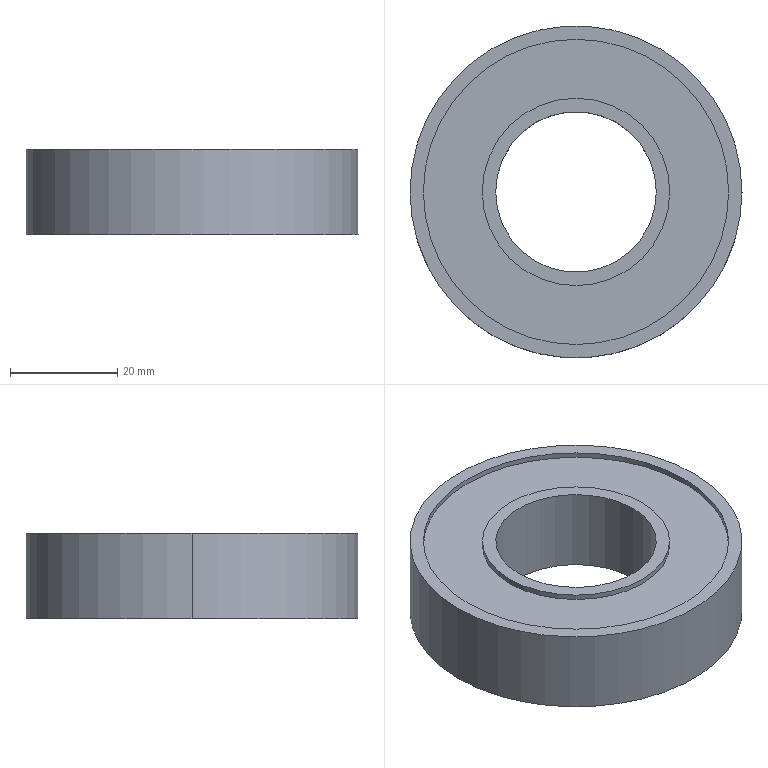Component | SolidWorks | 6206Bearing1-1 | 1 solid | 18 faces | box 62 x 62 x 16 mm | volume 33816 mm3 | cylinder 12 | plane 6 | commonest cylinder face diameters 35 x4 57 x4 30 x2 62 x2 | material AISI 1045 Steel, Cold Drawn
build123d program:
from build123d import *


with BuildPart() as part:
    # Sketch1 → Revolve1 (revolve)
    with BuildSketch(Plane(origin=(0, 0, 0), x_dir=(0, 0, -1), z_dir=(1, 0, 0)), mode=Mode.PRIVATE) as revolve1_sk:
        Polygon((-8, 15), (8, 15), (8, 17.5), (7, 17.5), (7, 28.5), (8, 28.5), (8, 31), (-8, 31), (-8, 28.5), (-7, 28.5), (-7, 17.5), (-8, 17.5), align=None)
    revolve(revolve1_sk.sketch.rotate(Axis((0, 0, -24.266), (0, 0, 1)), 90), axis=Axis((0, 0, -24.266), (0, 0, 1)))


solid = part.part

# Placed as in the assembly
solid = solid.moved(Location((-84.74, 1020.354, 45), (0, 0, 0)))
STEP:
#1=COLOUR_RGB('',0.7922,0.8196,0.9333);
#2=FILL_AREA_STYLE_COLOUR('',#1);
#3=FILL_AREA_STYLE('',(#2));
#4=SURFACE_STYLE_FILL_AREA(#3);
#5=SURFACE_SIDE_STYLE('',(#4));
#6=SURFACE_STYLE_USAGE(.BOTH.,#5);
#7=PRESENTATION_STYLE_ASSIGNMENT((#6));
#8=CARTESIAN_POINT('',(-2.746,40.171,2.087));
#9=VERTEX_POINT('',#8);
#10=CARTESIAN_POINT('',(-3.927,40.171,2.087));
#11=VERTEX_POINT('',#10);
#12=CARTESIAN_POINT('',(-3.336,40.171,2.087));
#13=DIRECTION('',(0.,-0.,-1.));
#14=DIRECTION('',(-1.,0.,0.));
#15=AXIS2_PLACEMENT_3D('',#12,#13,#14);
#16=CIRCLE('',#15,0.5906);
#17=EDGE_CURVE('',#9,#11,#16,.T.);
#18=ORIENTED_EDGE('',*,*,#17,.F.);
#19=CARTESIAN_POINT('',(-2.746,40.171,1.457));
#20=VERTEX_POINT('',#19);
#21=CARTESIAN_POINT('',(-2.746,40.171,0.8163));
#22=DIRECTION('',(0.,-0.,-1.));
#23=VECTOR('',#22,39.37);
#24=LINE('',#21,#23);
#25=EDGE_CURVE('',#9,#20,#24,.T.);
#26=ORIENTED_EDGE('',*,*,#25,.T.);
#27=CARTESIAN_POINT('',(-3.927,40.171,1.457));
#28=VERTEX_POINT('',#27);
#29=CARTESIAN_POINT('',(-3.336,40.171,1.457));
#30=DIRECTION('',(0.,-0.,-1.));
#31=DIRECTION('',(-1.,0.,0.));
#32=AXIS2_PLACEMENT_3D('',#29,#30,#31);
#33=CIRCLE('',#32,0.5906);
#34=EDGE_CURVE('',#20,#28,#33,.T.);
#35=ORIENTED_EDGE('',*,*,#34,.T.);
#36=CARTESIAN_POINT('',(-3.927,40.171,0.8163));
#37=DIRECTION('',(0.,-0.,-1.));
#38=VECTOR('',#37,39.37);
#39=LINE('',#36,#38);
#40=EDGE_CURVE('',#11,#28,#39,.T.);
#41=ORIENTED_EDGE('',*,*,#40,.F.);
#42=EDGE_LOOP('',(#18,#26,#35,#41));
#43=FACE_OUTER_BOUND('',#42,.T.);
#44=CARTESIAN_POINT('',(-3.336,40.171,0.8163));
#45=DIRECTION('',(0.,-0.,-1.));
#46=DIRECTION('',(-1.,0.,0.));
#47=AXIS2_PLACEMENT_3D('',#44,#45,#46);
#48=CYLINDRICAL_SURFACE('',#47,0.5906);
#49=ADVANCED_FACE('',(#43),#48,.F.);
#50=CARTESIAN_POINT('',(-4.025,40.171,2.087));
#51=VERTEX_POINT('',#50);
#52=CARTESIAN_POINT('',(-2.647,40.171,2.087));
#53=VERTEX_POINT('',#52);
#54=CARTESIAN_POINT('',(-3.336,40.171,2.087));
#55=DIRECTION('',(0.,-0.,-1.));
#56=DIRECTION('',(-1.,0.,0.));
#57=AXIS2_PLACEMENT_3D('',#54,#55,#56);
#58=CIRCLE('',#57,0.689);
#59=EDGE_CURVE('',#51,#53,#58,.T.);
#60=ORIENTED_EDGE('',*,*,#59,.T.);
#61=CARTESIAN_POINT('',(-2.647,40.171,2.047));
#62=VERTEX_POINT('',#61);
#63=CARTESIAN_POINT('',(-2.647,40.171,0.8163));
#64=DIRECTION('',(0.,-0.,-1.));
#65=VECTOR('',#64,39.37);
#66=LINE('',#63,#65);
#67=EDGE_CURVE('',#53,#62,#66,.T.);
#68=ORIENTED_EDGE('',*,*,#67,.T.);
#69=CARTESIAN_POINT('',(-4.025,40.171,2.047));
#70=VERTEX_POINT('',#69);
#71=CARTESIAN_POINT('',(-3.336,40.171,2.047));
#72=DIRECTION('',(0.,-0.,-1.));
#73=DIRECTION('',(-1.,0.,0.));
#74=AXIS2_PLACEMENT_3D('',#71,#72,#73);
#75=CIRCLE('',#74,0.689);
#76=EDGE_CURVE('',#70,#62,#75,.T.);
#77=ORIENTED_EDGE('',*,*,#76,.F.);
#78=CARTESIAN_POINT('',(-4.025,40.171,0.8163));
#79=DIRECTION('',(0.,-0.,-1.));
#80=VECTOR('',#79,39.37);
#81=LINE('',#78,#80);
#82=EDGE_CURVE('',#51,#70,#81,.T.);
#83=ORIENTED_EDGE('',*,*,#82,.F.);
#84=EDGE_LOOP('',(#60,#68,#77,#83));
#85=FACE_OUTER_BOUND('',#84,.T.);
#86=CARTESIAN_POINT('',(-3.336,40.171,0.8163));
#87=DIRECTION('',(0.,-0.,-1.));
#88=DIRECTION('',(-1.,0.,0.));
#89=AXIS2_PLACEMENT_3D('',#86,#87,#88);
#90=CYLINDRICAL_SURFACE('',#89,0.689);
#91=ADVANCED_FACE('',(#85),#90,.T.);
#92=CARTESIAN_POINT('',(-2.214,40.171,2.087));
#93=VERTEX_POINT('',#92);
#94=CARTESIAN_POINT('',(-4.458,40.171,2.087));
#95=VERTEX_POINT('',#94);
#96=CARTESIAN_POINT('',(-3.336,40.171,2.087));
#97=DIRECTION('',(0.,-0.,-1.));
#98=DIRECTION('',(-1.,0.,0.));
#99=AXIS2_PLACEMENT_3D('',#96,#97,#98);
#100=CIRCLE('',#99,1.122);
#101=EDGE_CURVE('',#93,#95,#100,.T.);
#102=ORIENTED_EDGE('',*,*,#101,.F.);
#103=CARTESIAN_POINT('',(-2.214,40.171,2.047));
#104=VERTEX_POINT('',#103);
#105=CARTESIAN_POINT('',(-2.214,40.171,0.8163));
#106=DIRECTION('',(0.,-0.,-1.));
#107=VECTOR('',#106,39.37);
#108=LINE('',#105,#107);
#109=EDGE_CURVE('',#93,#104,#108,.T.);
#110=ORIENTED_EDGE('',*,*,#109,.T.);
#111=CARTESIAN_POINT('',(-4.458,40.171,2.047));
#112=VERTEX_POINT('',#111);
#113=CARTESIAN_POINT('',(-3.336,40.171,2.047));
#114=DIRECTION('',(0.,-0.,-1.));
#115=DIRECTION('',(-1.,0.,0.));
#116=AXIS2_PLACEMENT_3D('',#113,#114,#115);
#117=CIRCLE('',#116,1.122);
#118=EDGE_CURVE('',#104,#112,#117,.T.);
#119=ORIENTED_EDGE('',*,*,#118,.T.);
#120=CARTESIAN_POINT('',(-4.458,40.171,0.8163));
#121=DIRECTION('',(0.,-0.,-1.));
#122=VECTOR('',#121,39.37);
#123=LINE('',#120,#122);
#124=EDGE_CURVE('',#95,#112,#123,.T.);
#125=ORIENTED_EDGE('',*,*,#124,.F.);
#126=EDGE_LOOP('',(#102,#110,#119,#125));
#127=FACE_OUTER_BOUND('',#126,.T.);
#128=CARTESIAN_POINT('',(-3.336,40.171,0.8163));
#129=DIRECTION('',(0.,-0.,-1.));
#130=DIRECTION('',(-1.,0.,0.));
#131=AXIS2_PLACEMENT_3D('',#128,#129,#130);
#132=CYLINDRICAL_SURFACE('',#131,1.122);
#133=ADVANCED_FACE('',(#127),#132,.F.);
#134=CARTESIAN_POINT('',(-4.557,40.171,2.087));
#135=VERTEX_POINT('',#134);
#136=CARTESIAN_POINT('',(-2.116,40.171,2.087));
#137=VERTEX_POINT('',#136);
#138=CARTESIAN_POINT('',(-3.336,40.171,2.087));
#139=DIRECTION('',(0.,-0.,-1.));
#140=DIRECTION('',(-1.,0.,0.));
#141=AXIS2_PLACEMENT_3D('',#138,#139,#140);
#142=CIRCLE('',#141,1.22);
#143=EDGE_CURVE('',#135,#137,#142,.T.);
#144=ORIENTED_EDGE('',*,*,#143,.T.);
#145=CARTESIAN_POINT('',(-2.116,40.171,1.457));
#146=VERTEX_POINT('',#145);
#147=CARTESIAN_POINT('',(-2.116,40.171,0.8163));
#148=DIRECTION('',(0.,-0.,-1.));
#149=VECTOR('',#148,39.37);
#150=LINE('',#147,#149);
#151=EDGE_CURVE('',#137,#146,#150,.T.);
#152=ORIENTED_EDGE('',*,*,#151,.T.);
#153=CARTESIAN_POINT('',(-4.557,40.171,1.457));
#154=VERTEX_POINT('',#153);
#155=CARTESIAN_POINT('',(-3.336,40.171,1.457));
#156=DIRECTION('',(0.,-0.,-1.));
#157=DIRECTION('',(-1.,0.,0.));
#158=AXIS2_PLACEMENT_3D('',#155,#156,#157);
#159=CIRCLE('',#158,1.22);
#160=EDGE_CURVE('',#154,#146,#159,.T.);
#161=ORIENTED_EDGE('',*,*,#160,.F.);
#162=CARTESIAN_POINT('',(-4.557,40.171,0.8163));
#163=DIRECTION('',(0.,-0.,-1.));
#164=VECTOR('',#163,39.37);
#165=LINE('',#162,#164);
#166=EDGE_CURVE('',#135,#154,#165,.T.);
#167=ORIENTED_EDGE('',*,*,#166,.F.);
#168=EDGE_LOOP('',(#144,#152,#161,#167));
#169=FACE_OUTER_BOUND('',#168,.T.);
#170=CARTESIAN_POINT('',(-3.336,40.171,0.8163));
#171=DIRECTION('',(0.,-0.,-1.));
#172=DIRECTION('',(-1.,0.,0.));
#173=AXIS2_PLACEMENT_3D('',#170,#171,#172);
#174=CYLINDRICAL_SURFACE('',#173,1.22);
#175=ADVANCED_FACE('',(#169),#174,.T.);
#176=CARTESIAN_POINT('',(-2.214,40.171,1.496));
#177=VERTEX_POINT('',#176);
#178=CARTESIAN_POINT('',(-4.458,40.171,1.496));
#179=VERTEX_POINT('',#178);
#180=CARTESIAN_POINT('',(-3.336,40.171,1.496));
#181=DIRECTION('',(0.,-0.,-1.));
#182=DIRECTION('',(-1.,0.,0.));
#183=AXIS2_PLACEMENT_3D('',#180,#181,#182);
#184=CIRCLE('',#183,1.122);
#185=EDGE_CURVE('',#177,#179,#184,.T.);
#186=ORIENTED_EDGE('',*,*,#185,.F.);
#187=CARTESIAN_POINT('',(-2.214,40.171,1.457));
#188=VERTEX_POINT('',#187);
#189=CARTESIAN_POINT('',(-2.214,40.171,0.8163));
#190=DIRECTION('',(0.,-0.,-1.));
#191=VECTOR('',#190,39.37);
#192=LINE('',#189,#191);
#193=EDGE_CURVE('',#177,#188,#192,.T.);
#194=ORIENTED_EDGE('',*,*,#193,.T.);
#195=CARTESIAN_POINT('',(-4.458,40.171,1.457));
#196=VERTEX_POINT('',#195);
#197=CARTESIAN_POINT('',(-3.336,40.171,1.457));
#198=DIRECTION('',(0.,-0.,-1.));
#199=DIRECTION('',(-1.,0.,0.));
#200=AXIS2_PLACEMENT_3D('',#197,#198,#199);
#201=CIRCLE('',#200,1.122);
#202=EDGE_CURVE('',#188,#196,#201,.T.);
#203=ORIENTED_EDGE('',*,*,#202,.T.);
#204=CARTESIAN_POINT('',(-4.458,40.171,0.8163));
#205=DIRECTION('',(0.,-0.,-1.));
#206=VECTOR('',#205,39.37);
#207=LINE('',#204,#206);
#208=EDGE_CURVE('',#179,#196,#207,.T.);
#209=ORIENTED_EDGE('',*,*,#208,.F.);
#210=EDGE_LOOP('',(#186,#194,#203,#209));
#211=FACE_OUTER_BOUND('',#210,.T.);
#212=CARTESIAN_POINT('',(-3.336,40.171,0.8163));
#213=DIRECTION('',(0.,-0.,-1.));
#214=DIRECTION('',(-1.,0.,0.));
#215=AXIS2_PLACEMENT_3D('',#212,#213,#214);
#216=CYLINDRICAL_SURFACE('',#215,1.122);
#217=ADVANCED_FACE('',(#211),#216,.F.);
#218=CARTESIAN_POINT('',(-4.025,40.171,1.496));
#219=VERTEX_POINT('',#218);
#220=CARTESIAN_POINT('',(-2.647,40.171,1.496));
#221=VERTEX_POINT('',#220);
#222=CARTESIAN_POINT('',(-3.336,40.171,1.496));
#223=DIRECTION('',(0.,-0.,-1.));
#224=DIRECTION('',(-1.,0.,0.));
#225=AXIS2_PLACEMENT_3D('',#222,#223,#224);
#226=CIRCLE('',#225,0.689);
#227=EDGE_CURVE('',#219,#221,#226,.T.);
#228=ORIENTED_EDGE('',*,*,#227,.T.);
#229=CARTESIAN_POINT('',(-2.647,40.171,1.457));
#230=VERTEX_POINT('',#229);
#231=CARTESIAN_POINT('',(-2.647,40.171,0.8163));
#232=DIRECTION('',(0.,-0.,-1.));
#233=VECTOR('',#232,39.37);
#234=LINE('',#231,#233);
#235=EDGE_CURVE('',#221,#230,#234,.T.);
#236=ORIENTED_EDGE('',*,*,#235,.T.);
#237=CARTESIAN_POINT('',(-4.025,40.171,1.457));
#238=VERTEX_POINT('',#237);
#239=CARTESIAN_POINT('',(-3.336,40.171,1.457));
#240=DIRECTION('',(0.,-0.,-1.));
#241=DIRECTION('',(-1.,0.,0.));
#242=AXIS2_PLACEMENT_3D('',#239,#240,#241);
#243=CIRCLE('',#242,0.689);
#244=EDGE_CURVE('',#238,#230,#243,.T.);
#245=ORIENTED_EDGE('',*,*,#244,.F.);
#246=CARTESIAN_POINT('',(-4.025,40.171,0.8163));
#247=DIRECTION('',(0.,-0.,-1.));
#248=VECTOR('',#247,39.37);
#249=LINE('',#246,#248);
#250=EDGE_CURVE('',#219,#238,#249,.T.);
#251=ORIENTED_EDGE('',*,*,#250,.F.);
#252=EDGE_LOOP('',(#228,#236,#245,#251));
#253=FACE_OUTER_BOUND('',#252,.T.);
#254=CARTESIAN_POINT('',(-3.336,40.171,0.8163));
#255=DIRECTION('',(0.,-0.,-1.));
#256=DIRECTION('',(-1.,0.,0.));
#257=AXIS2_PLACEMENT_3D('',#254,#255,#256);
#258=CYLINDRICAL_SURFACE('',#257,0.689);
#259=ADVANCED_FACE('',(#253),#258,.T.);
#260=ORIENTED_EDGE('',*,*,#244,.T.);
#261=CARTESIAN_POINT('',(-3.336,40.171,1.457));
#262=DIRECTION('',(0.,-0.,-1.));
#263=DIRECTION('',(-1.,0.,0.));
#264=AXIS2_PLACEMENT_3D('',#261,#262,#263);
#265=CIRCLE('',#264,0.689);
#266=EDGE_CURVE('',#230,#238,#265,.T.);
#267=ORIENTED_EDGE('',*,*,#266,.T.);
#268=EDGE_LOOP('',(#260,#267));
#269=FACE_OUTER_BOUND('',#268,.T.);
#270=CARTESIAN_POINT('',(-3.336,40.171,1.457));
#271=DIRECTION('',(0.,-0.,-1.));
#272=DIRECTION('',(-1.,0.,0.));
#273=AXIS2_PLACEMENT_3D('',#270,#271,#272);
#274=CIRCLE('',#273,0.5906);
#275=EDGE_CURVE('',#28,#20,#274,.T.);
#276=ORIENTED_EDGE('',*,*,#275,.F.);
#277=ORIENTED_EDGE('',*,*,#34,.F.);
#278=EDGE_LOOP('',(#276,#277));
#279=FACE_BOUND('',#278,.T.);
#280=CARTESIAN_POINT('',(-3.336,40.762,1.457));
#281=DIRECTION('',(-0.,-0.,-1.));
#282=DIRECTION('',(-1.,0.,0.));
#283=AXIS2_PLACEMENT_3D('',#280,#281,#282);
#284=PLANE('',#283);
#285=ADVANCED_FACE('',(#269,#279),#284,.T.);
#286=ORIENTED_EDGE('',*,*,#235,.F.);
#287=CARTESIAN_POINT('',(-3.336,40.171,1.496));
#288=DIRECTION('',(0.,-0.,-1.));
#289=DIRECTION('',(-1.,0.,0.));
#290=AXIS2_PLACEMENT_3D('',#287,#288,#289);
#291=CIRCLE('',#290,0.689);
#292=EDGE_CURVE('',#221,#219,#291,.T.);
#293=ORIENTED_EDGE('',*,*,#292,.T.);
#294=ORIENTED_EDGE('',*,*,#250,.T.);
#295=ORIENTED_EDGE('',*,*,#266,.F.);
#296=EDGE_LOOP('',(#286,#293,#294,#295));
#297=FACE_OUTER_BOUND('',#296,.T.);
#298=CARTESIAN_POINT('',(-3.336,40.171,0.8163));
#299=DIRECTION('',(0.,-0.,-1.));
#300=DIRECTION('',(-1.,0.,0.));
#301=AXIS2_PLACEMENT_3D('',#298,#299,#300);
#302=CYLINDRICAL_SURFACE('',#301,0.689);
#303=ADVANCED_FACE('',(#297),#302,.T.);
#304=CARTESIAN_POINT('',(-3.336,40.171,1.496));
#305=DIRECTION('',(0.,-0.,-1.));
#306=DIRECTION('',(-1.,0.,0.));
#307=AXIS2_PLACEMENT_3D('',#304,#305,#306);
#308=CIRCLE('',#307,1.122);
#309=EDGE_CURVE('',#179,#177,#308,.T.);
#310=ORIENTED_EDGE('',*,*,#309,.T.);
#311=ORIENTED_EDGE('',*,*,#185,.T.);
#312=EDGE_LOOP('',(#310,#311));
#313=FACE_OUTER_BOUND('',#312,.T.);
#314=ORIENTED_EDGE('',*,*,#227,.F.);
#315=ORIENTED_EDGE('',*,*,#292,.F.);
#316=EDGE_LOOP('',(#314,#315));
#317=FACE_BOUND('',#316,.T.);
#318=CARTESIAN_POINT('',(-3.336,40.86,1.496));
#319=DIRECTION('',(-0.,-0.,-1.));
#320=DIRECTION('',(-1.,0.,0.));
#321=AXIS2_PLACEMENT_3D('',#318,#319,#320);
#322=PLANE('',#321);
#323=ADVANCED_FACE('',(#313,#317),#322,.T.);
#324=ORIENTED_EDGE('',*,*,#193,.F.);
#325=ORIENTED_EDGE('',*,*,#309,.F.);
#326=ORIENTED_EDGE('',*,*,#208,.T.);
#327=CARTESIAN_POINT('',(-3.336,40.171,1.457));
#328=DIRECTION('',(0.,-0.,-1.));
#329=DIRECTION('',(-1.,0.,0.));
#330=AXIS2_PLACEMENT_3D('',#327,#328,#329);
#331=CIRCLE('',#330,1.122);
#332=EDGE_CURVE('',#196,#188,#331,.T.);
#333=ORIENTED_EDGE('',*,*,#332,.T.);
#334=EDGE_LOOP('',(#324,#325,#326,#333));
#335=FACE_OUTER_BOUND('',#334,.T.);
#336=CARTESIAN_POINT('',(-3.336,40.171,0.8163));
#337=DIRECTION('',(0.,-0.,-1.));
#338=DIRECTION('',(-1.,0.,0.));
#339=AXIS2_PLACEMENT_3D('',#336,#337,#338);
#340=CYLINDRICAL_SURFACE('',#339,1.122);
#341=ADVANCED_FACE('',(#335),#340,.F.);
#342=ORIENTED_EDGE('',*,*,#160,.T.);
#343=CARTESIAN_POINT('',(-3.336,40.171,1.457));
#344=DIRECTION('',(0.,-0.,-1.));
#345=DIRECTION('',(-1.,0.,0.));
#346=AXIS2_PLACEMENT_3D('',#343,#344,#345);
#347=CIRCLE('',#346,1.22);
#348=EDGE_CURVE('',#146,#154,#347,.T.);
#349=ORIENTED_EDGE('',*,*,#348,.T.);
#350=EDGE_LOOP('',(#342,#349));
#351=FACE_OUTER_BOUND('',#350,.T.);
#352=ORIENTED_EDGE('',*,*,#332,.F.);
#353=ORIENTED_EDGE('',*,*,#202,.F.);
#354=EDGE_LOOP('',(#352,#353));
#355=FACE_BOUND('',#354,.T.);
#356=CARTESIAN_POINT('',(-3.336,41.293,1.457));
#357=DIRECTION('',(-0.,-0.,-1.));
#358=DIRECTION('',(-1.,0.,0.));
#359=AXIS2_PLACEMENT_3D('',#356,#357,#358);
#360=PLANE('',#359);
#361=ADVANCED_FACE('',(#351,#355),#360,.T.);
#362=ORIENTED_EDGE('',*,*,#151,.F.);
#363=CARTESIAN_POINT('',(-3.336,40.171,2.087));
#364=DIRECTION('',(0.,-0.,-1.));
#365=DIRECTION('',(-1.,0.,0.));
#366=AXIS2_PLACEMENT_3D('',#363,#364,#365);
#367=CIRCLE('',#366,1.22);
#368=EDGE_CURVE('',#137,#135,#367,.T.);
#369=ORIENTED_EDGE('',*,*,#368,.T.);
#370=ORIENTED_EDGE('',*,*,#166,.T.);
#371=ORIENTED_EDGE('',*,*,#348,.F.);
#372=EDGE_LOOP('',(#362,#369,#370,#371));
#373=FACE_OUTER_BOUND('',#372,.T.);
#374=CARTESIAN_POINT('',(-3.336,40.171,0.8163));
#375=DIRECTION('',(0.,-0.,-1.));
#376=DIRECTION('',(-1.,0.,0.));
#377=AXIS2_PLACEMENT_3D('',#374,#375,#376);
#378=CYLINDRICAL_SURFACE('',#377,1.22);
#379=ADVANCED_FACE('',(#373),#378,.T.);
#380=CARTESIAN_POINT('',(-3.336,40.171,2.087));
#381=DIRECTION('',(0.,-0.,-1.));
#382=DIRECTION('',(-1.,0.,0.));
#383=AXIS2_PLACEMENT_3D('',#380,#381,#382);
#384=CIRCLE('',#383,1.122);
#385=EDGE_CURVE('',#95,#93,#384,.T.);
#386=ORIENTED_EDGE('',*,*,#385,.T.);
#387=ORIENTED_EDGE('',*,*,#101,.T.);
#388=EDGE_LOOP('',(#386,#387));
#389=FACE_BOUND('',#388,.T.);
#390=ORIENTED_EDGE('',*,*,#143,.F.);
#391=ORIENTED_EDGE('',*,*,#368,.F.);
#392=EDGE_LOOP('',(#390,#391));
#393=FACE_OUTER_BOUND('',#392,.T.);
#394=CARTESIAN_POINT('',(-3.336,41.293,2.087));
#395=DIRECTION('',(0.,0.,1.));
#396=DIRECTION('',(1.,-0.,-0.));
#397=AXIS2_PLACEMENT_3D('',#394,#395,#396);
#398=PLANE('',#397);
#399=ADVANCED_FACE('',(#389,#393),#398,.T.);
#400=ORIENTED_EDGE('',*,*,#109,.F.);
#401=ORIENTED_EDGE('',*,*,#385,.F.);
#402=ORIENTED_EDGE('',*,*,#124,.T.);
#403=CARTESIAN_POINT('',(-3.336,40.171,2.047));
#404=DIRECTION('',(0.,-0.,-1.));
#405=DIRECTION('',(-1.,0.,0.));
#406=AXIS2_PLACEMENT_3D('',#403,#404,#405);
#407=CIRCLE('',#406,1.122);
#408=EDGE_CURVE('',#112,#104,#407,.T.);
#409=ORIENTED_EDGE('',*,*,#408,.T.);
#410=EDGE_LOOP('',(#400,#401,#402,#409));
#411=FACE_OUTER_BOUND('',#410,.T.);
#412=CARTESIAN_POINT('',(-3.336,40.171,0.8163));
#413=DIRECTION('',(0.,-0.,-1.));
#414=DIRECTION('',(-1.,0.,0.));
#415=AXIS2_PLACEMENT_3D('',#412,#413,#414);
#416=CYLINDRICAL_SURFACE('',#415,1.122);
#417=ADVANCED_FACE('',(#411),#416,.F.);
#418=ORIENTED_EDGE('',*,*,#76,.T.);
#419=CARTESIAN_POINT('',(-3.336,40.171,2.047));
#420=DIRECTION('',(0.,-0.,-1.));
#421=DIRECTION('',(-1.,0.,0.));
#422=AXIS2_PLACEMENT_3D('',#419,#420,#421);
#423=CIRCLE('',#422,0.689);
#424=EDGE_CURVE('',#62,#70,#423,.T.);
#425=ORIENTED_EDGE('',*,*,#424,.T.);
#426=EDGE_LOOP('',(#418,#425));
#427=FACE_BOUND('',#426,.T.);
#428=ORIENTED_EDGE('',*,*,#408,.F.);
#429=ORIENTED_EDGE('',*,*,#118,.F.);
#430=EDGE_LOOP('',(#428,#429));
#431=FACE_OUTER_BOUND('',#430,.T.);
#432=CARTESIAN_POINT('',(-3.336,40.86,2.047));
#433=DIRECTION('',(0.,0.,1.));
#434=DIRECTION('',(1.,-0.,-0.));
#435=AXIS2_PLACEMENT_3D('',#432,#433,#434);
#436=PLANE('',#435);
#437=ADVANCED_FACE('',(#427,#431),#436,.T.);
#438=ORIENTED_EDGE('',*,*,#67,.F.);
#439=CARTESIAN_POINT('',(-3.336,40.171,2.087));
#440=DIRECTION('',(0.,-0.,-1.));
#441=DIRECTION('',(-1.,0.,0.));
#442=AXIS2_PLACEMENT_3D('',#439,#440,#441);
#443=CIRCLE('',#442,0.689);
#444=EDGE_CURVE('',#53,#51,#443,.T.);
#445=ORIENTED_EDGE('',*,*,#444,.T.);
#446=ORIENTED_EDGE('',*,*,#82,.T.);
#447=ORIENTED_EDGE('',*,*,#424,.F.);
#448=EDGE_LOOP('',(#438,#445,#446,#447));
#449=FACE_OUTER_BOUND('',#448,.T.);
#450=CARTESIAN_POINT('',(-3.336,40.171,0.8163));
#451=DIRECTION('',(0.,-0.,-1.));
#452=DIRECTION('',(-1.,0.,0.));
#453=AXIS2_PLACEMENT_3D('',#450,#451,#452);
#454=CYLINDRICAL_SURFACE('',#453,0.689);
#455=ADVANCED_FACE('',(#449),#454,.T.);
#456=CARTESIAN_POINT('',(-3.336,40.171,2.087));
#457=DIRECTION('',(0.,-0.,-1.));
#458=DIRECTION('',(-1.,0.,0.));
#459=AXIS2_PLACEMENT_3D('',#456,#457,#458);
#460=CIRCLE('',#459,0.5906);
#461=EDGE_CURVE('',#11,#9,#460,.T.);
#462=ORIENTED_EDGE('',*,*,#461,.T.);
#463=ORIENTED_EDGE('',*,*,#17,.T.);
#464=EDGE_LOOP('',(#462,#463));
#465=FACE_BOUND('',#464,.T.);
#466=ORIENTED_EDGE('',*,*,#59,.F.);
#467=ORIENTED_EDGE('',*,*,#444,.F.);
#468=EDGE_LOOP('',(#466,#467));
#469=FACE_OUTER_BOUND('',#468,.T.);
#470=CARTESIAN_POINT('',(-3.336,40.762,2.087));
#471=DIRECTION('',(0.,0.,1.));
#472=DIRECTION('',(1.,-0.,-0.));
#473=AXIS2_PLACEMENT_3D('',#470,#471,#472);
#474=PLANE('',#473);
#475=ADVANCED_FACE('',(#465,#469),#474,.T.);
#476=ORIENTED_EDGE('',*,*,#25,.F.);
#477=ORIENTED_EDGE('',*,*,#461,.F.);
#478=ORIENTED_EDGE('',*,*,#40,.T.);
#479=ORIENTED_EDGE('',*,*,#275,.T.);
#480=EDGE_LOOP('',(#476,#477,#478,#479));
#481=FACE_OUTER_BOUND('',#480,.T.);
#482=CARTESIAN_POINT('',(-3.336,40.171,0.8163));
#483=DIRECTION('',(0.,-0.,-1.));
#484=DIRECTION('',(-1.,0.,0.));
#485=AXIS2_PLACEMENT_3D('',#482,#483,#484);
#486=CYLINDRICAL_SURFACE('',#485,0.5906);
#487=ADVANCED_FACE('',(#481),#486,.F.);
#488=CLOSED_SHELL('',(#49,#91,#133,#175,#217,#259,#285,#303,#323,#341,#361,#379,#399,#417,#437,#455,#475,#487));
#489=MANIFOLD_SOLID_BREP('',#488);
#490=STYLED_ITEM('',(#7),#489);
#491=(LENGTH_UNIT()NAMED_UNIT(*)SI_UNIT($,.METRE.));
#492=LENGTH_MEASURE_WITH_UNIT(LENGTH_MEASURE(0.0254),#491);
#493=DIMENSIONAL_EXPONENTS(1.,0.,0.,0.,0.,0.,0.);
#494=(CONVERSION_BASED_UNIT('',#492)LENGTH_UNIT()NAMED_UNIT(#493));
#495=UNCERTAINTY_MEASURE_WITH_UNIT(LENGTH_MEASURE(0.00001),#494,'','');
#496=(NAMED_UNIT(*)PLANE_ANGLE_UNIT()SI_UNIT($,.RADIAN.));
#497=(NAMED_UNIT(*)SI_UNIT($,.STERADIAN.)SOLID_ANGLE_UNIT());
#498=(GEOMETRIC_REPRESENTATION_CONTEXT(3)GLOBAL_UNCERTAINTY_ASSIGNED_CONTEXT((#495))GLOBAL_UNIT_ASSIGNED_CONTEXT((#494,#496,#497))REPRESENTATION_CONTEXT('',''));
#499=MECHANICAL_DESIGN_GEOMETRIC_PRESENTATION_REPRESENTATION('',(#490),#498);
#500=CARTESIAN_POINT('',(0.,0.,0.));
#501=DIRECTION('',(0.,0.,1.));
#502=DIRECTION('',(1.,0.,0.));
#503=AXIS2_PLACEMENT_3D('',#500,#501,#502);
#504=(LENGTH_UNIT()NAMED_UNIT(*)SI_UNIT($,.METRE.));
#505=LENGTH_MEASURE_WITH_UNIT(LENGTH_MEASURE(0.0254),#504);
#506=DIMENSIONAL_EXPONENTS(1.,0.,0.,0.,0.,0.,0.);
#507=(CONVERSION_BASED_UNIT('',#505)LENGTH_UNIT()NAMED_UNIT(#506));
#508=UNCERTAINTY_MEASURE_WITH_UNIT(LENGTH_MEASURE(0.00001),#507,'','');
#509=(NAMED_UNIT(*)PLANE_ANGLE_UNIT()SI_UNIT($,.RADIAN.));
#510=(NAMED_UNIT(*)SI_UNIT($,.STERADIAN.)SOLID_ANGLE_UNIT());
#511=(GEOMETRIC_REPRESENTATION_CONTEXT(3)GLOBAL_UNCERTAINTY_ASSIGNED_CONTEXT((#508))GLOBAL_UNIT_ASSIGNED_CONTEXT((#507,#509,#510))REPRESENTATION_CONTEXT('',''));
#512=ADVANCED_BREP_SHAPE_REPRESENTATION('',(#489,#503),#511);
#513=PRESENTATION_LAYER_ASSIGNMENT('','',(#490));